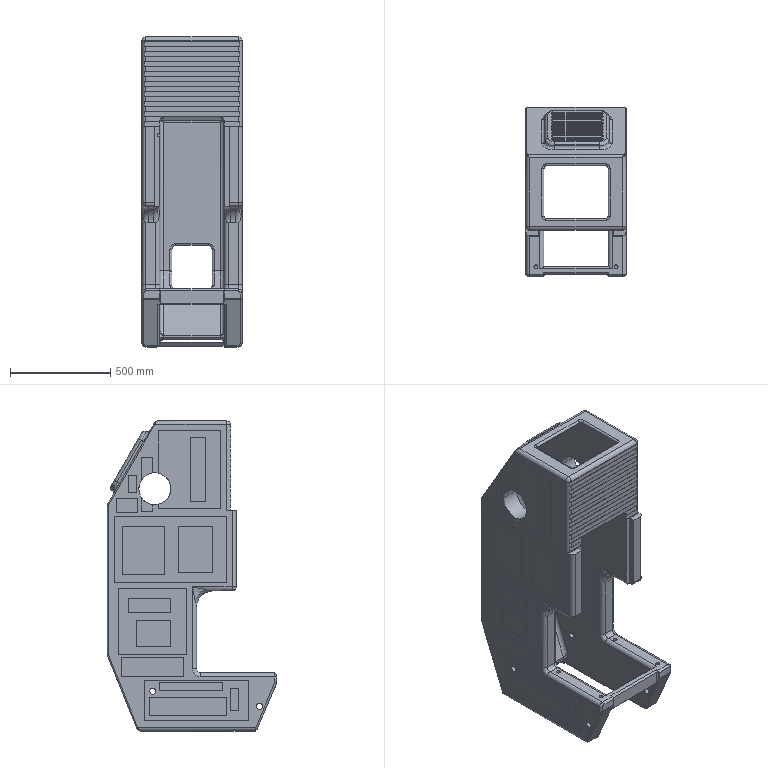Component | SolidWorks | Frame-1 | 1 solid | 530 faces | volume 188268771 mm3 | plane 296 | cylinder 148 | spline 52 | torus 26 | sphere 4 | cone 4 | commonest cylinder face diameters 40 x45 20 x30 30 x18 19 x18 6 x18 10 x11 160.02 x4 16.2 x2